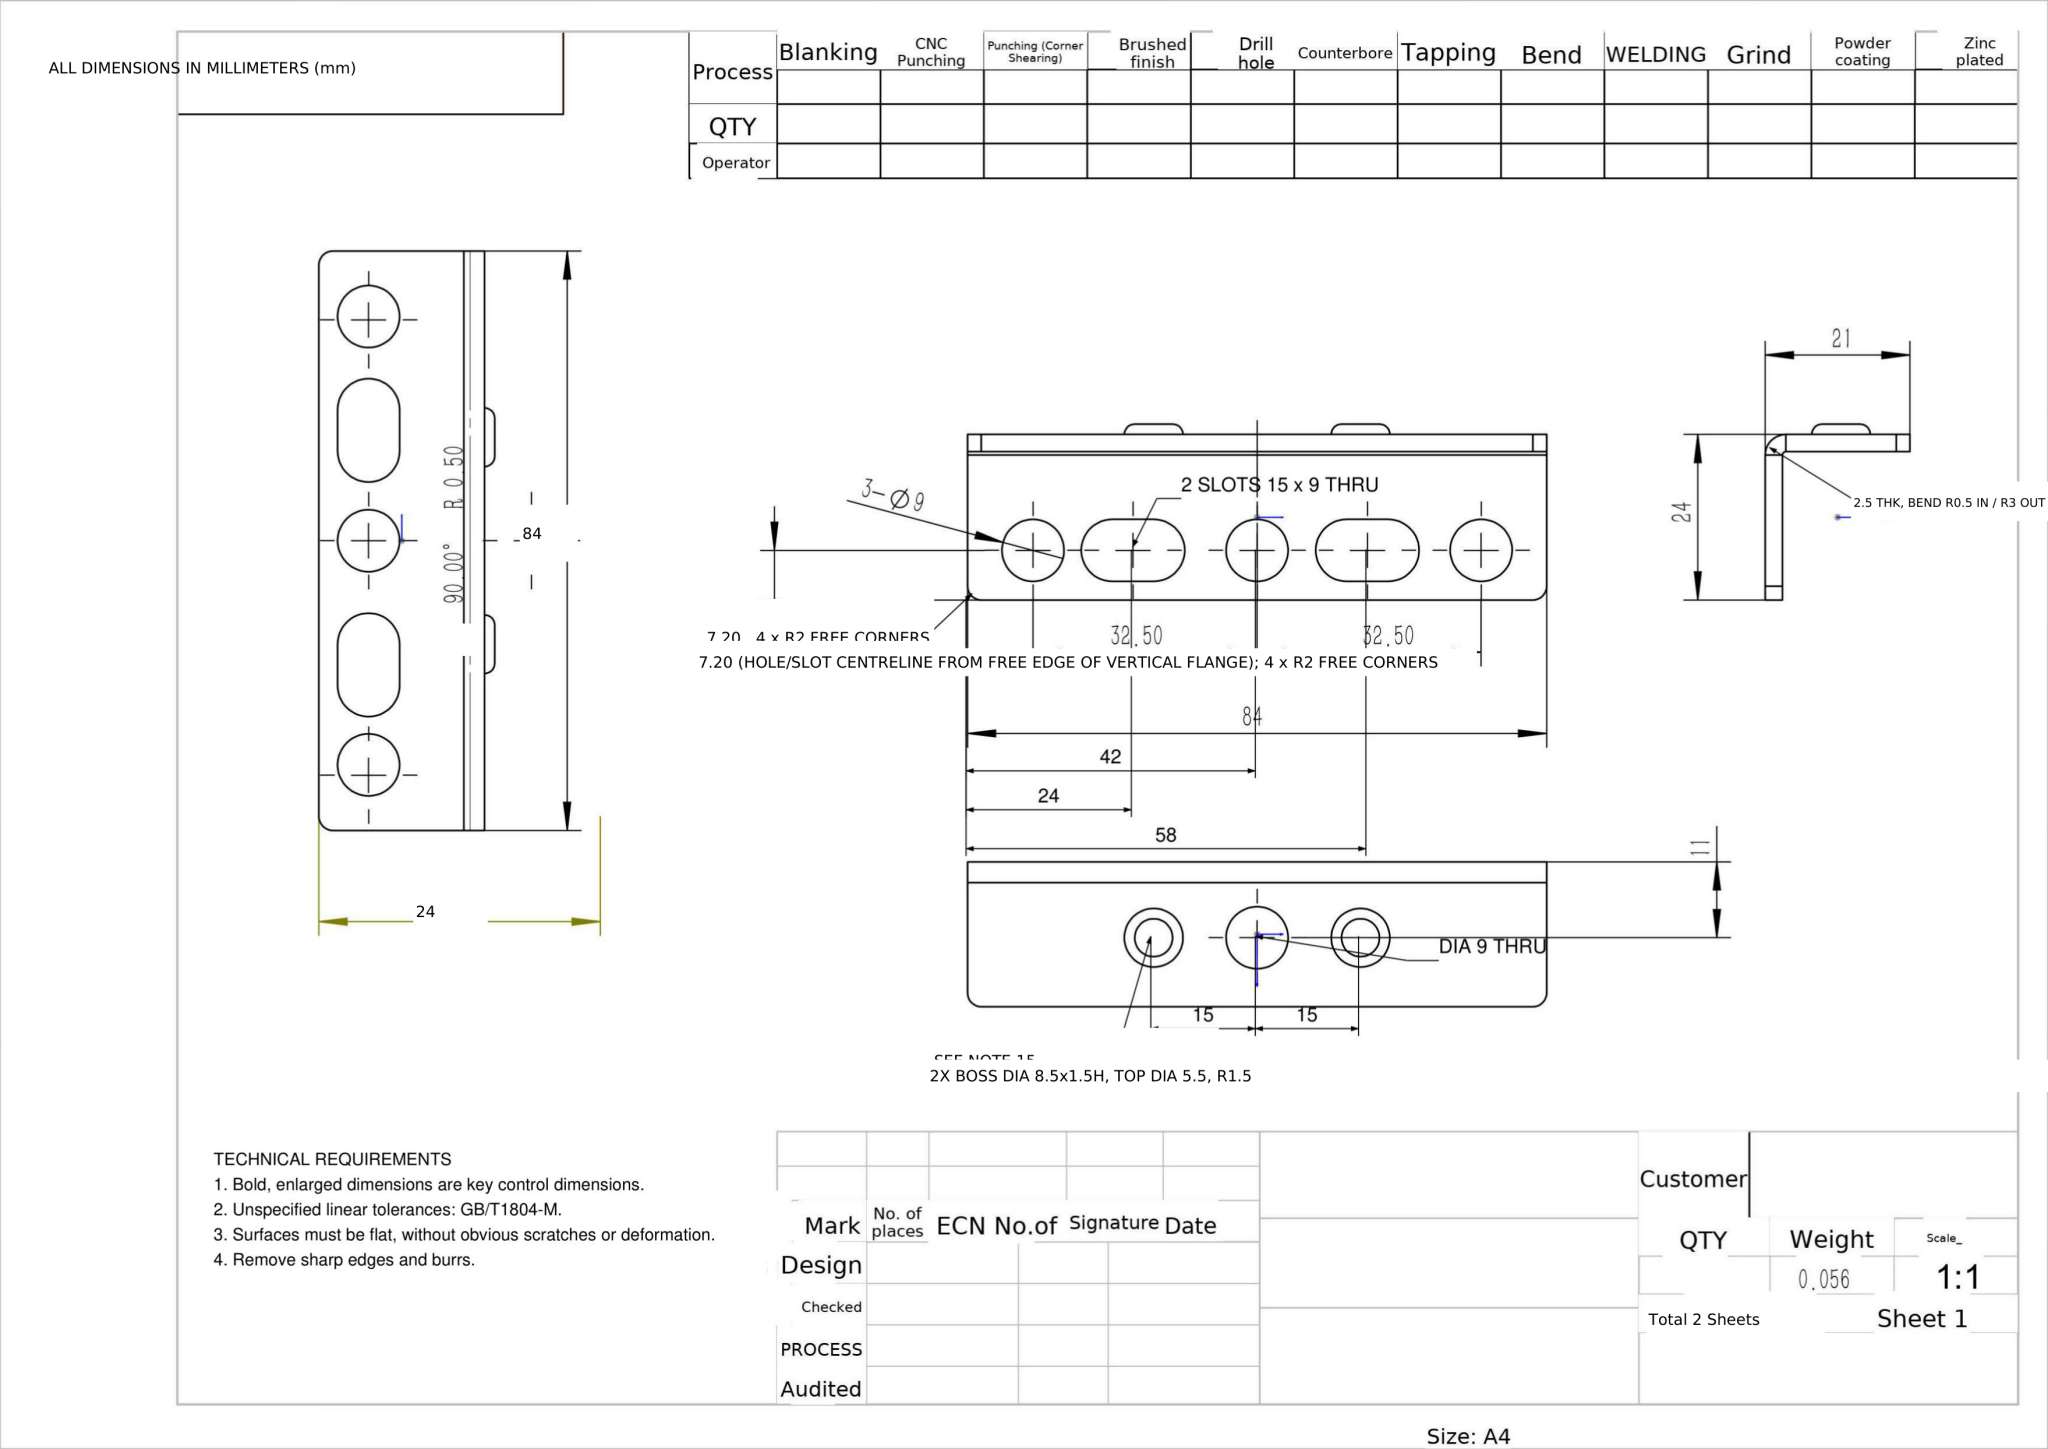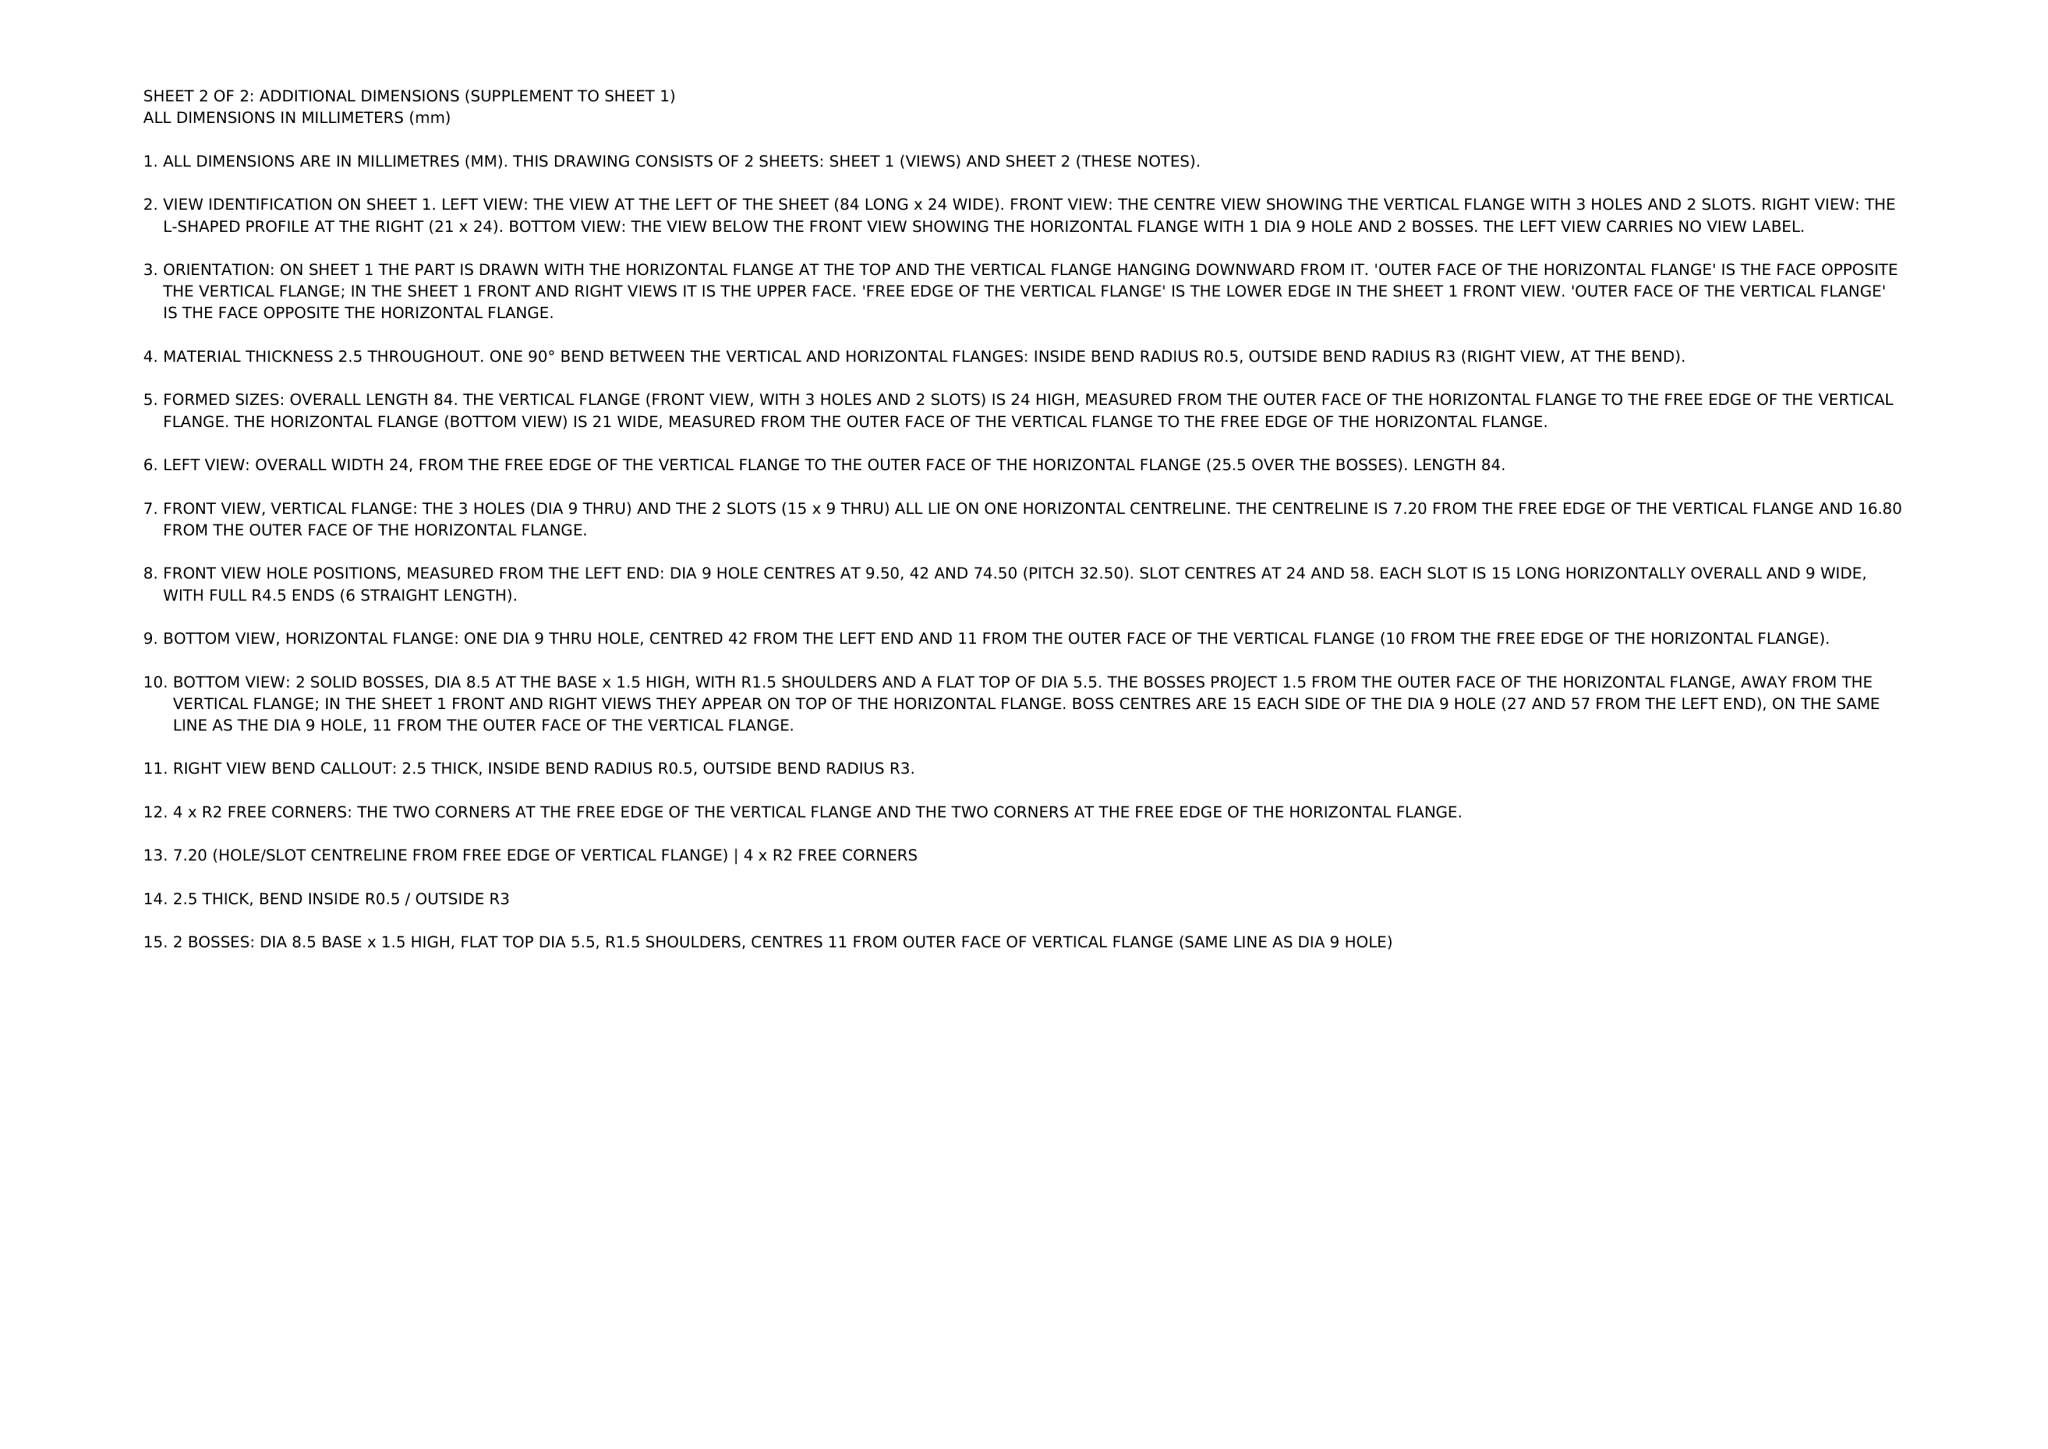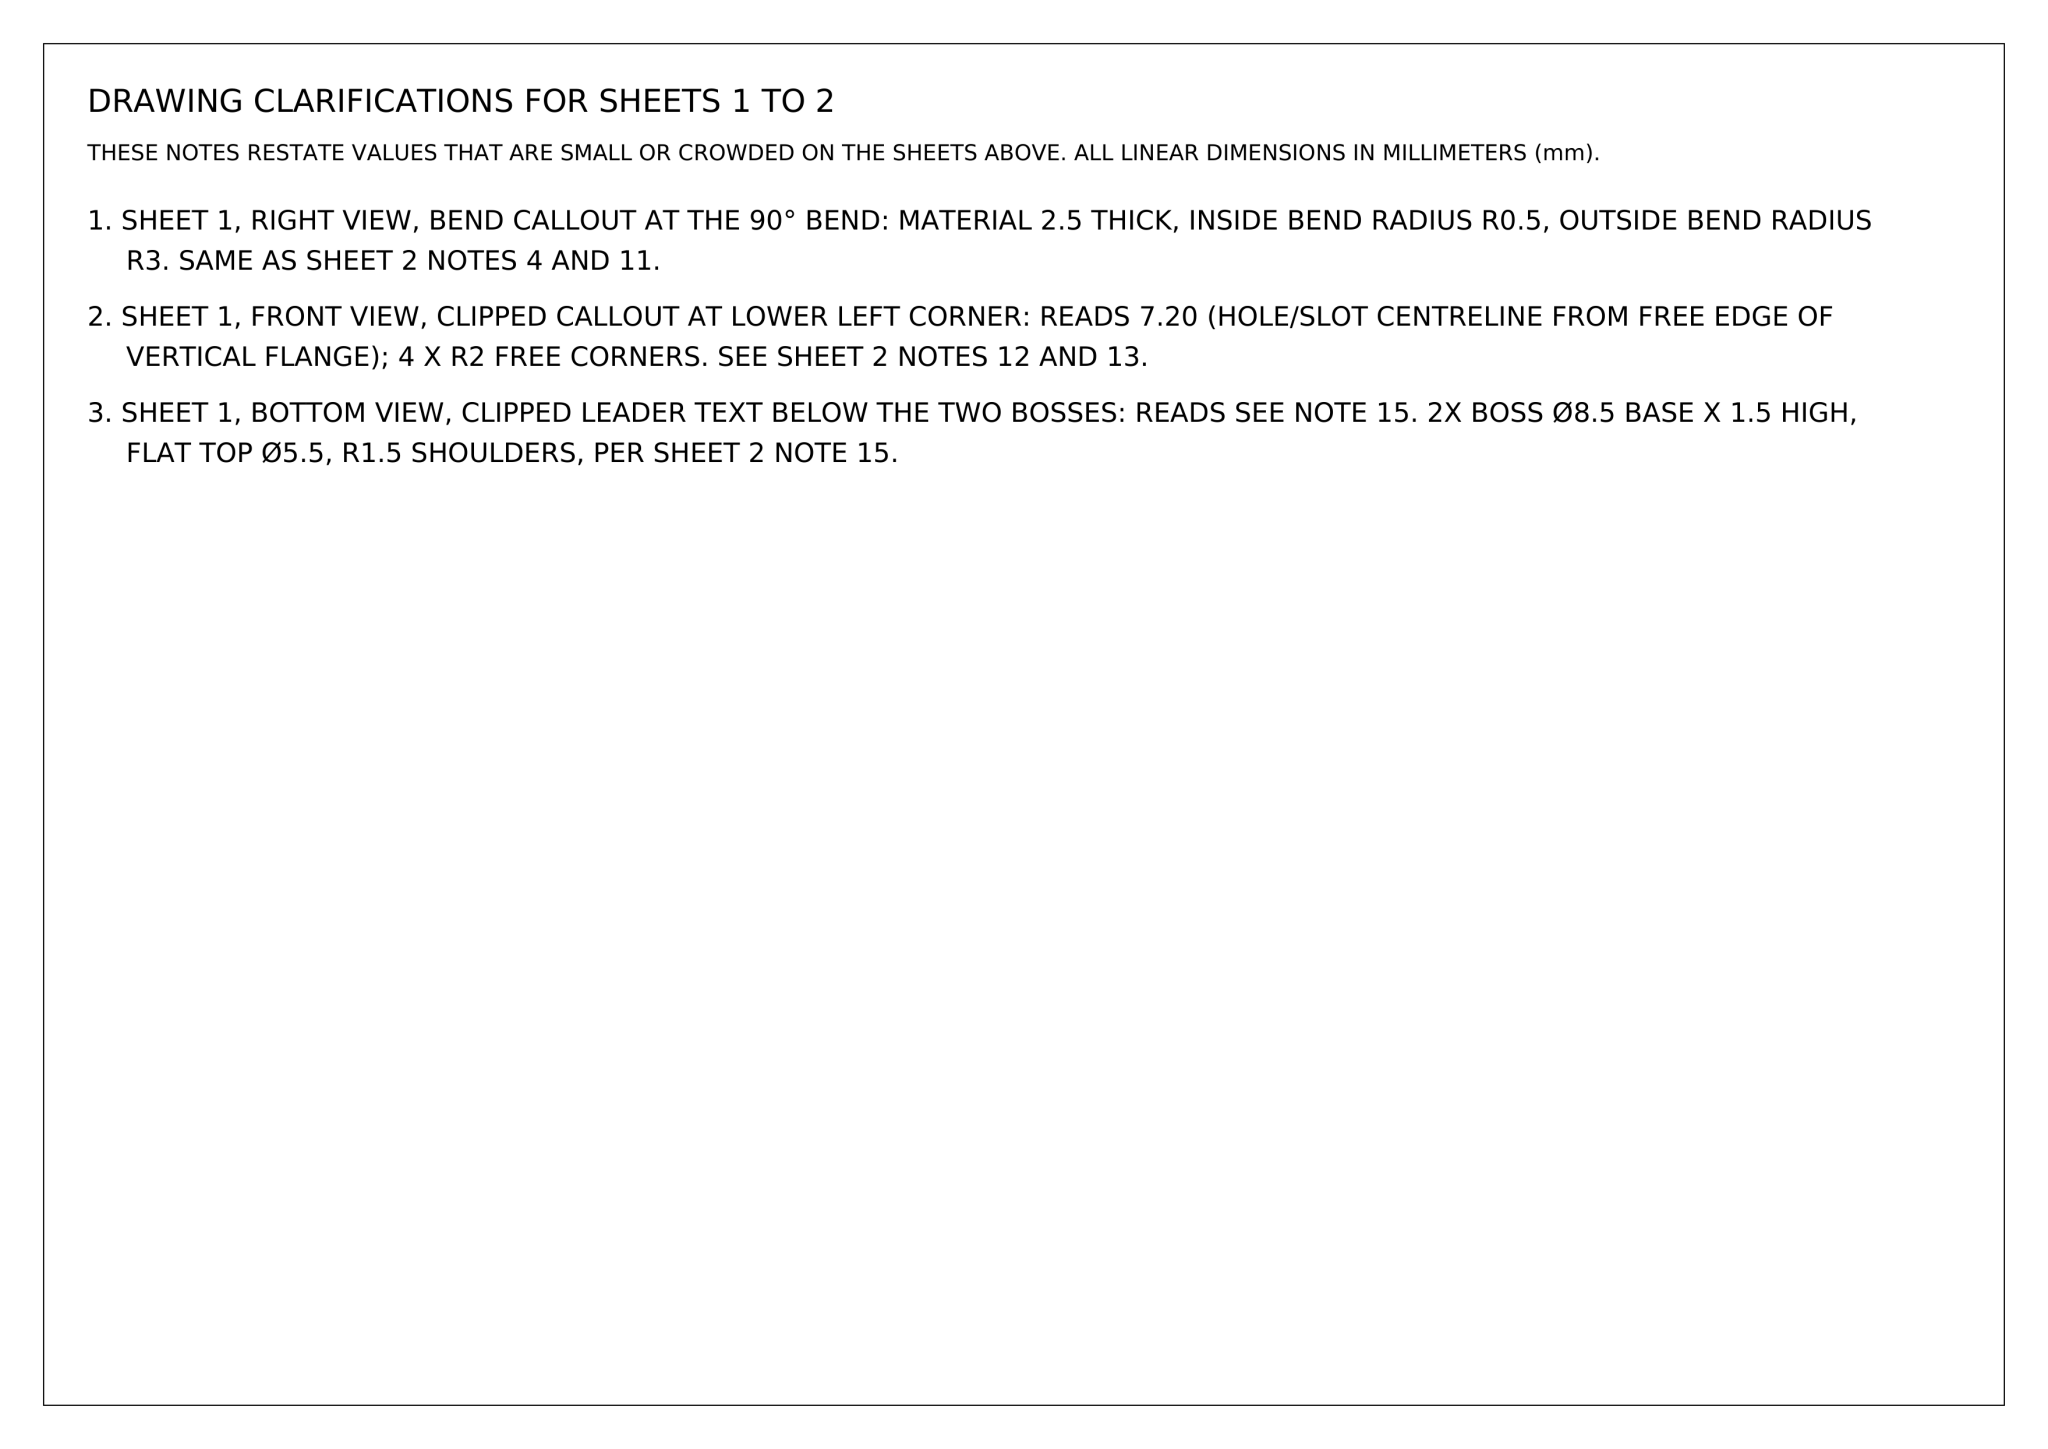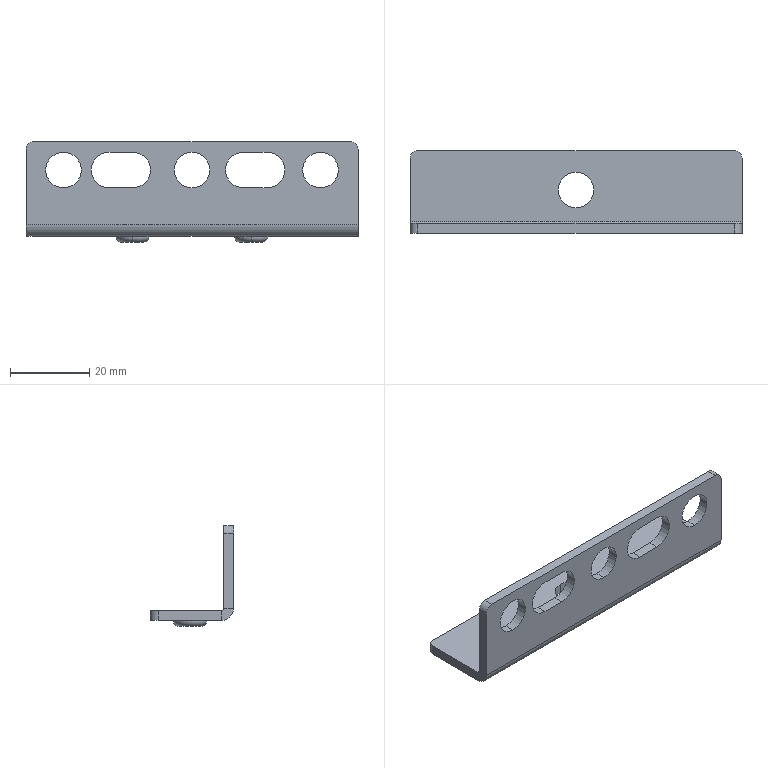Part | NX | mm | 1 solid | 40 faces | box 84 x 21 x 25.5 mm | volume 7681 mm3 | cylinder 18 | plane 18 | torus 4 | commonest cylinder face diameters 9 x12 4 x4 6 x1 1 x1